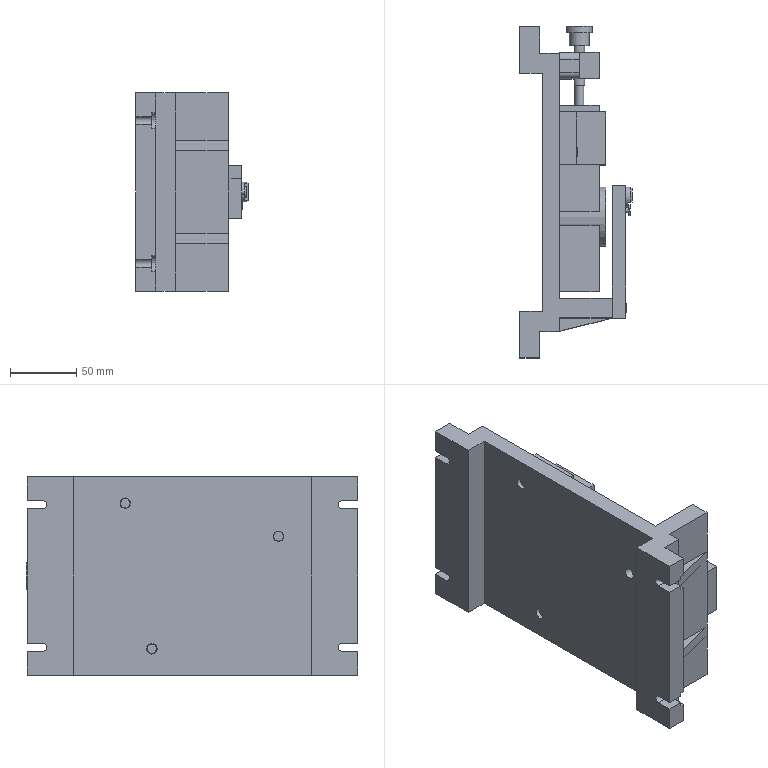Assembly | NX | mm | 20 component files | 20 solids | 345 faces | box 85 x 250.73 x 150 mm | volume 1099999 mm3 | plane 194 | cylinder 81 | cone 46 | torus 24 | commonest cylinder face diameters 8 x33 13 x18 10 x12 12 x4 6 x4 15 x3 4 x2 5 x2
Bill of materials:
unnamed part 1 | 1 |  | Stepped, axially symmetric pin with a thin large-diameter head flange, a shorter collar of medium diameter, a long shank, and a short step down to a slightly smaller-diameter end section.
unnamed part 2 | 2 |  | Plain solid cylinder with small chamfers on both ends.
unnamed part 3 | 1 |  | Block made of a bar with fully rounded ends (stadium outline) and a rectangular boss sticking out from one side at mid-length. There is one through hole near each rounded end and a cross hole through the middle section.
unnamed part 4 | 1 |  | Short solid cylinder, slightly shorter than its diameter, with one small hole near the edge of one end face.
unnamed part 5 | 2 |  | Socket-head screw-like part: cylindrical head with a hexagonal socket and rounded top edge, a fillet under the head, and a plain cylindrical shank with a chamfered tip.
unnamed part 6 | 1 |  | Socket-head screw-like part: cylindrical head with a hexagonal socket and rounded top edge, a fillet under the head, and a relatively long plain cylindrical shank with a chamfered tip.
unnamed part 7 | 1 |  | Slotted-head pin or screw-like part: short cylindrical head with a chamfered outer edge and a straight slot cut right across it, on a plain cylindrical shank with a chamfered end.
unnamed part 8 | 1 |  | Rectangular block with a V-shaped notch cut fully through its thickness along one long face. The bottom of the V has a small flat-bottomed rectangular relief slot.
unnamed part 9 | 1 |  | Hat-section (offset U-shaped) bracket: a thin-walled U-shaped middle section, with thicker end tabs pointing outward at both ends. Each tab has two through holes of different sizes.
unnamed part 10 | 1 |  | Flanged bushing-like part with a central through bore. It has a cylindrical body with a chamfered end and a larger chamfered flange. One side of the flange has a partial-depth flat or step cut into it.
unnamed part 11 | 1 |  | Flat rectangular plate with three through holes: two of different sizes at one end and one larger hole at the other end. There is also a small blind hole next to the single hole.
unnamed part 12 | 1 |  | Rectangular block with a V-shaped notch cut through its thickness on one side, with a flat-bottomed rectangular relief at the bottom of the V. There are two through holes of different sizes near the corners on the opposite side.
unnamed part 13 | 1 |  | Rectangular plate-like block with stepped flanges along both long edges, giving a stepped, roughly Z/C-shaped profile in end view; one edge carries an angled, tapered lip. The main face has several small holes and four open-ended slots on its short edges.
unnamed part 14 | 3 |  | Headed cylindrical fastener-like part: a plain cylindrical shank with a chamfered end and a larger cylindrical head with rounded edges and a hexagonal socket recess with a conical bottom.
unnamed part 15 | 1 |  | Plain solid cylinder (rod or pin) with small chamfers on both ends; the length is roughly five times the diameter.
unnamed part 16 | 1 |  | Plain solid cylinder (rod or pin) with small chamfers on both ends; it is shorter and stubbier than part-e711, with a length roughly four times the diameter.
Mates:
1. concentric | drill_jig_plate 1 edge | jig_body 1 edge
2. concentric | dowel_pin_8x30 1 edge | drill_jig_plate 1 edge
3. concentric | m8x20 1 edge | drill_jig_plate 1 edge
4. concentric | fixed_v_block 1 edge | jig_body 1 edge
5. concentric | dowel_pin_8x40 1 edge | fixed_v_block 1 edge
6. concentric | m8x30 3 edge | fixed_v_block 1 edge
7. touch align | handle_sleeve 1 face | jig_body 1 face
8. distance | handle_sleeve 1 face | fixed_v_block 1 face
9. touch align | handle_sleeve 1 face | fixed_v_block 1 face
10. concentric | drill_bushing 1 edge | drill_jig_plate 1 edge
11. touch align | screw 1 face | drill_bushing 1 face
12. touch align | movable_v_block 1 face | jig_body 1 face
13. distance | handle_sleeve 1 face | movable_v_block 1 face
14. touch align | handle_sleeve 1 face | movable_v_block 1 face
15. touch align | movable_base 1 face | jig_body 1 face
16. touch align | movable_base 1 face | movable_v_block 1 face
17. distance | movable_base 1 face | movable_v_block 1 face
18. concentric | m8x15 2 edge | movable_base 1 edge
19. concentric | m8x15 1 edge | movable_base 1 edge
20. concentric | dowel_pin_8x20 2 edge | movable_base 1 edge
21. concentric | dowel_pin_8x20 1 edge | movable_base 1 edge
22. concentric | handle 1 edge | movable_v_block 1 edge
23. align lock | fixed_base 1 face | handle 1 face
24. distance | fixed_base 1 face | handle 1 face
25. concentric | m8x30 2 edge | fixed_base 1 edge
26. concentric | m8x30 1 edge | fixed_base 1 edge